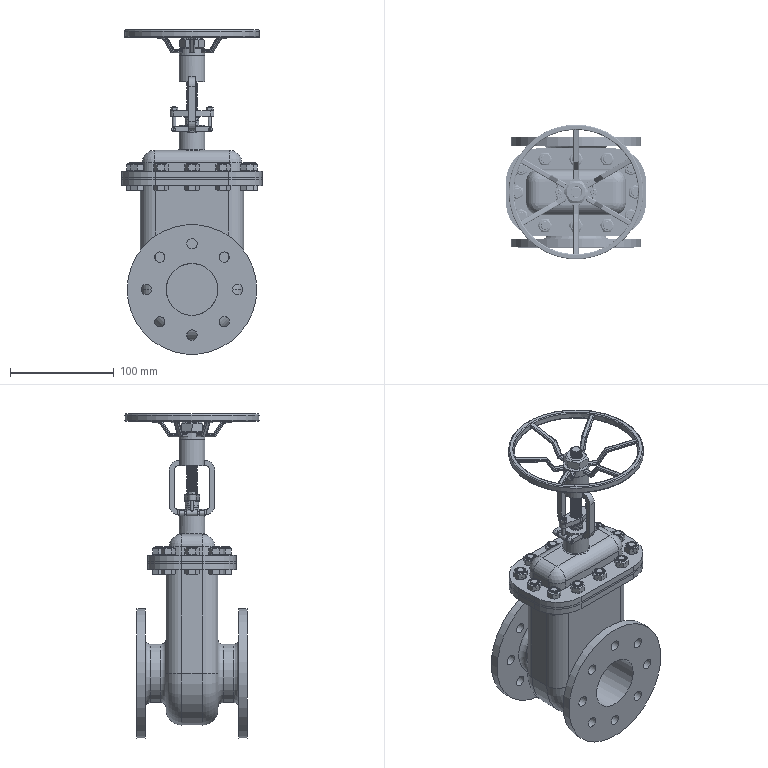Assembly | NX | mm | 37 component files | 37 solids | 1041 faces | box 135 x 130 x 312.5 mm | volume 588204 mm3 | cylinder 490 | plane 409 | spline 72 | cone 48 | torus 14 | sphere 8 | commonest cylinder face diameters 8 x134 10 x132 2 x72 3 x24 10.2 x22 24 x16 64 x12 18 x12
Bill of materials:
unnamed part 1 | 1 |  | Hollow flanged body. It has two opposed circular end flanges joined by a narrow central body, and a rounded-rectangle flange on top that is perpendicular to the end flanges.
unnamed part 2 | 1 |  | Thin circular disc with chamfered edges and a slender rod extending outward from one point on its rim. The rod is plain near the disc and has thread-like grooves over its outer portion.
unnamed part 3 | 1 |  | Flanged cover-like part. A flat rounded-rectangle flange carries a raised domed housing, and a cylindrical neck rises from the dome to a rectangular loop frame topped by a cylindrical boss.
unnamed part 4 | 2 |  | T-shaped part: a short hollow cylindrical cross-tube with a through-bore, and a perpendicular round rod attached at its mid-length with a thread-like grooved end.
unnamed part 5 | 12 |  | Hex-head bolt-like part with a chamfered hexagonal head, a plain cylindrical shank, and a short thread-like grooved section at the tip.
unnamed part 6 | 12 |  | Hexagonal nut-like part with chamfered corners on both faces and a central bore that has internal thread-like grooves. The bore is large relative to the hex size.
unnamed part 7 | 1 |  | Spoked wheel: a thin circular rim joined to a central hub by six evenly spaced spokes. Each spoke has a cranked (offset) profile, so the hub sits below the plane of the rim.
unnamed part 8 | 1 |  | Hexagonal nut-like part with corner chamfers on both faces and a central bore with internal thread-like grooves.
unnamed part 9 | 1 |  | Flat, diamond-shaped plate with rounded ends, a large central bore with internal thread-like grooves, and a small through-hole near each end.
unnamed part 10 | 2 |  | Plain solid cylindrical pin with small chamfers at both ends.
unnamed part 11 | 2 |  | Hexagonal nut-like part with corner chamfers on both faces and a central bore with internal thread-like grooves.
unnamed part 12 | 1 |  | Very thin flat sheet with a rounded-rectangle outline, a large rounded-rectangle central opening, and 12 small through-holes around the border.
Mates:
1. fix | valve_body 1 component
2. touch align | washer 1 face | valve_body 1 face
3. touch align | washer 1 face | valve_body 1 face
4. touch align | valve_body 1 face | washer 1 face
5. touch align | washer 1 face | top_cover 1 face
6. touch align | top_cover 1 face | valve_body 1 face
7. touch align | top_cover 1 face | valve_body 1 face
8. concentric | top_cover 1 edge | fastener 1 arc
9. parallel | fastener 1 face | top_cover 1 face
10. parallel | valve_cap 1 face | valve_body 1 face
11. touch align | valve_cap 1 face | top_cover 1 face
12. concentric | top_cover 1 edge | handwheel 1 edge
13. concentric | handwheel 1 edge | nut_M10 1 arc
14. concentric | nut_M8x6 12 edge | valve_body 1 edge
15. parallel | nut_M8x6 12 face | valve_body 1 face
16. concentric | nut_M8x6 11 edge | valve_body 1 edge
17. parallel | nut_M8x6 11 face | valve_body 1 face
18. concentric | valve_body 1 edge | nut_M8x6 10 edge
19. parallel | nut_M8x6 10 face | valve_body 1 face
20. concentric | valve_body 1 edge | nut_M8x6 9 edge
21. parallel | nut_M8x6 9 face | valve_body 1 face
22. concentric | nut_M8x6 8 edge | valve_body 1 edge
23. parallel | nut_M8x6 8 face | valve_body 1 face
24. concentric | valve_body 1 edge | nut_M8x6 7 edge
25. parallel | nut_M8x6 7 face | valve_body 1 face
26. concentric | nut_M8x6 6 edge | valve_body 1 edge
27. parallel | nut_M8x6 6 face | valve_body 1 face
28. concentric | valve_body 1 edge | nut_M8x6 5 edge
29. parallel | nut_M8x6 5 face | valve_body 1 face
30. concentric | valve_body 1 edge | nut_M8x6 4 edge
31. parallel | nut_M8x6 4 face | valve_body 1 face
32. concentric | valve_body 1 edge | nut_M8x6 3 edge
33. parallel | nut_M8x6 3 face | valve_body 1 face
34. concentric | nut_M8x6 2 edge | valve_body 1 edge
35. parallel | nut_M8x6 2 face | valve_body 1 face
36. concentric | nut_M8x6 1 edge | valve_body 1 edge
37. parallel | nut_M8x6 1 face | valve_body 1 face
38. parallel | nut_M8 12 face | top_cover 1 face
39. concentric | top_cover 1 edge | nut_M8 11 arc
40. parallel | nut_M8 11 face | top_cover 1 face
41. parallel | nut_M8 10 face | top_cover 1 face
42. concentric | top_cover 1 edge | nut_M8 9 arc
43. parallel | nut_M8 9 face | top_cover 1 face
44. concentric | top_cover 1 edge | nut_M8 8 arc
45. parallel | nut_M8 8 face | top_cover 1 face
46. concentric | top_cover 1 edge | nut_M8 7 arc
47. parallel | nut_M8 7 face | top_cover 1 face
48. parallel | nut_M8 6 face | top_cover 1 face
49. concentric | top_cover 1 edge | nut_M8 5 arc
50. parallel | nut_M8 5 face | top_cover 1 face
51. concentric | nut_M8 4 arc | top_cover 1 edge
52. parallel | nut_M8 4 face | top_cover 1 face
53. parallel | nut_M8 3 face | top_cover 1 face
54. concentric | nut_M8 2 arc | top_cover 1 edge
55. parallel | nut_M8 2 face | top_cover 1 face
56. concentric | top_cover 1 edge | nut_M8 1 arc
57. parallel | nut_M8 1 face | top_cover 1 face
58. concentric | connector 2 edge | top_cover 1 edge
59. concentric | connector 1 edge | top_cover 1 edge
60. touch align | locating_post 2 face | connector 1 face
61. center | locating_post 2 face | locating_post 2 face | top_cover 1 face | top_cover 1 face
62. parallel | locating_post 2 face | top_cover 1 face
63. touch align | locating_post 1 face | connector 2 face
64. touch align | locating_post 1 face | fastener 1 face
65. concentric | fastener 1 edge | nut_M3 2 arc
66. concentric | fastener 1 edge | nut_M3 1 arc
67. parallel | nut_M3 1 face | top_cover 1 face
68. parallel | nut_M3 2 face | top_cover 1 face